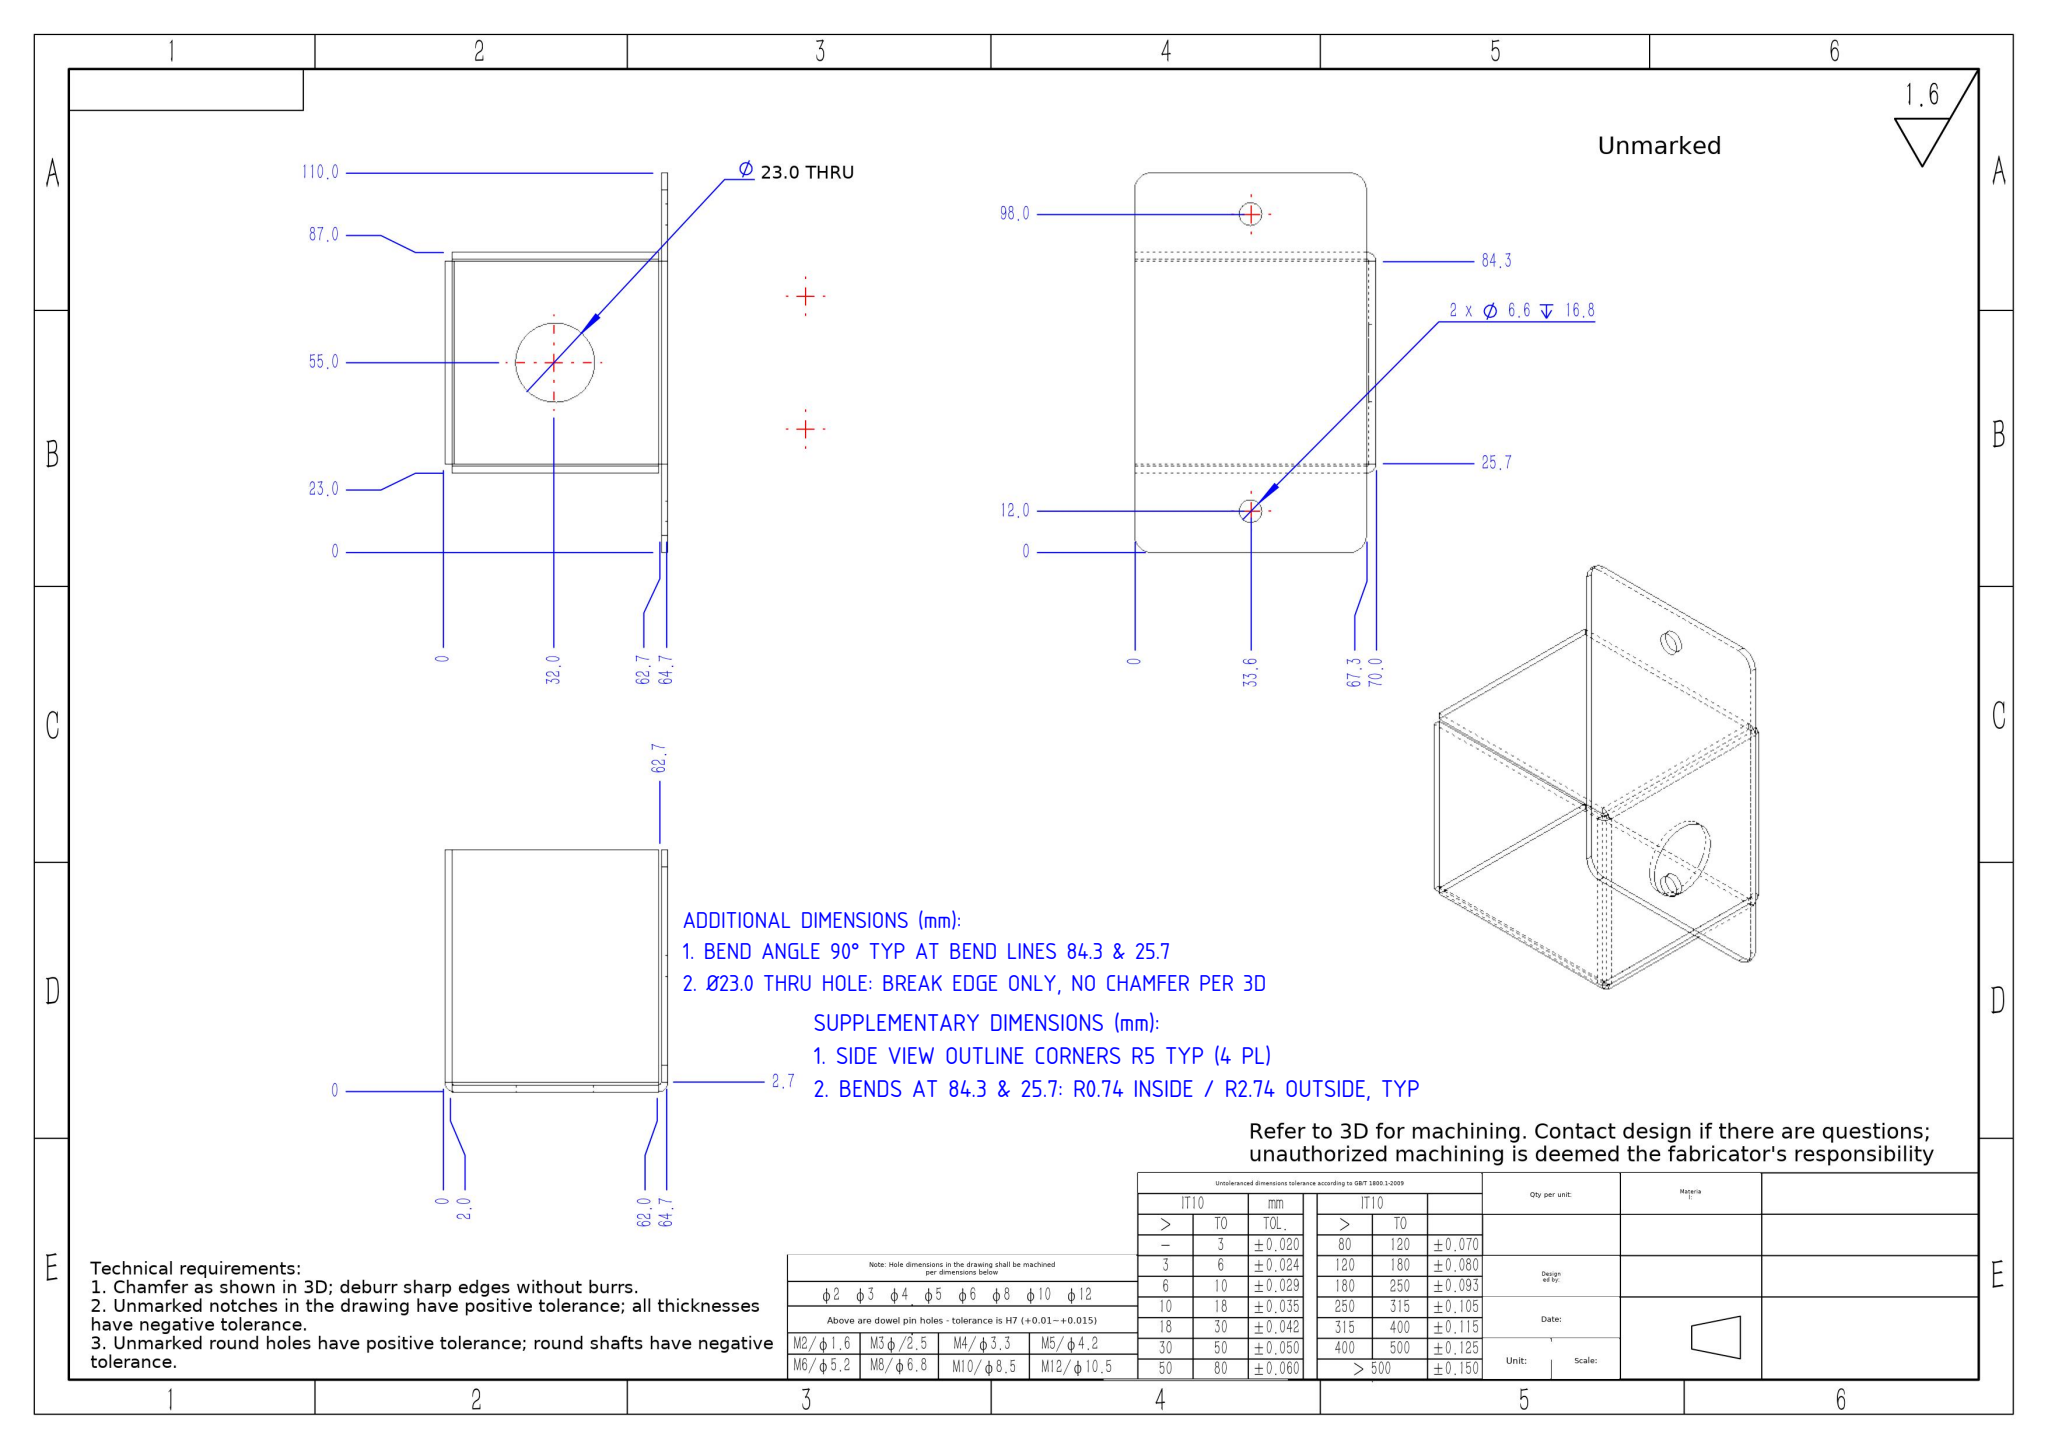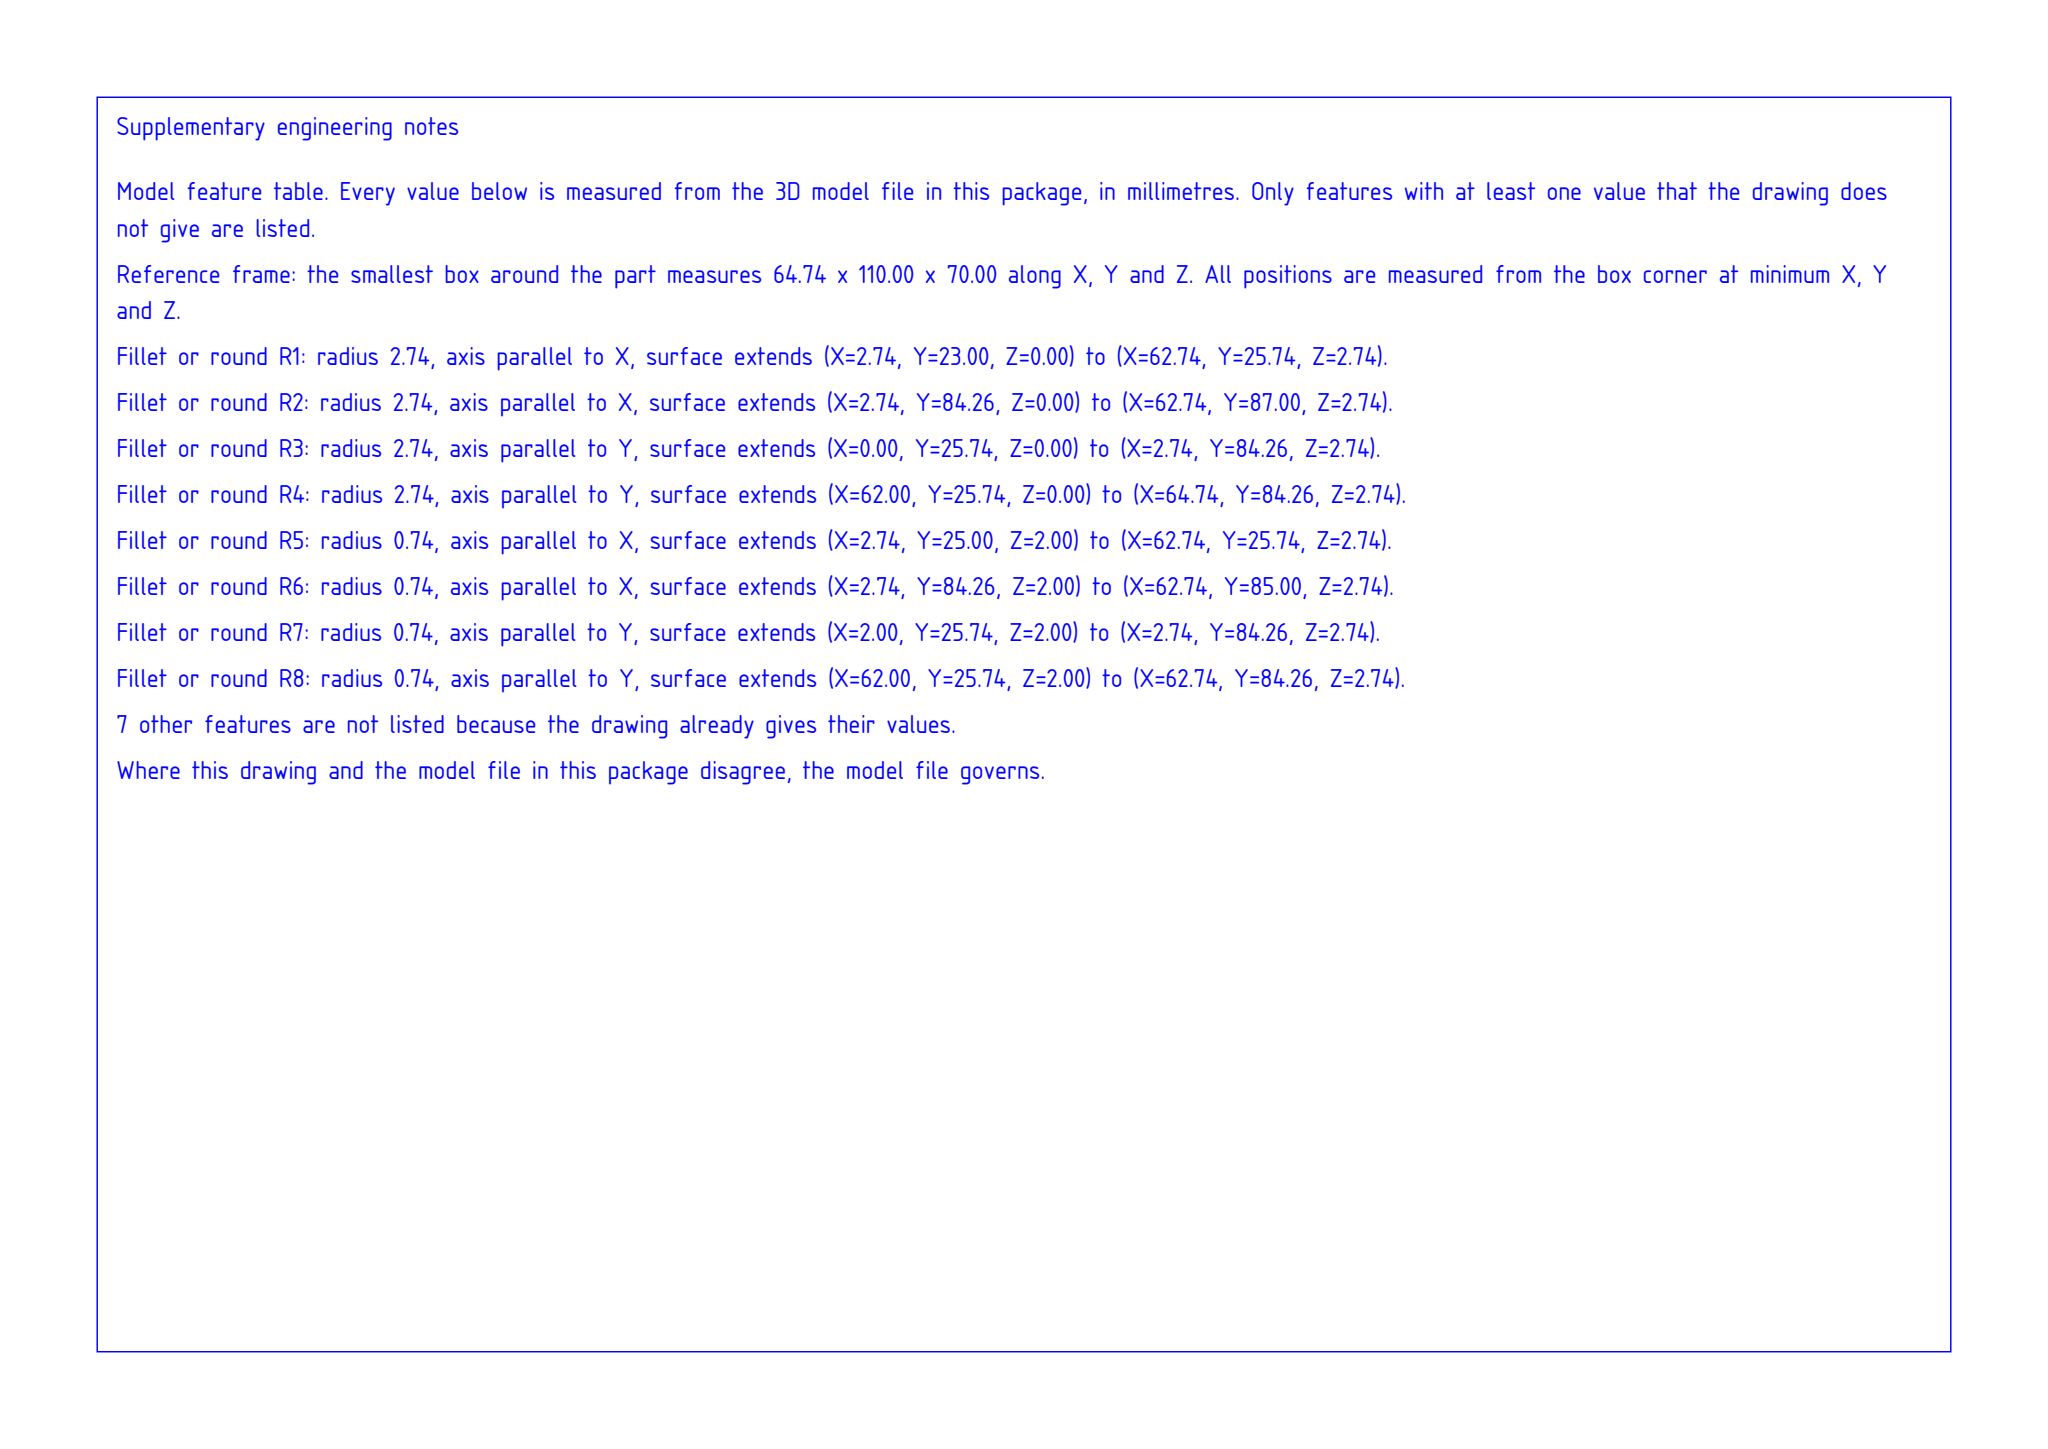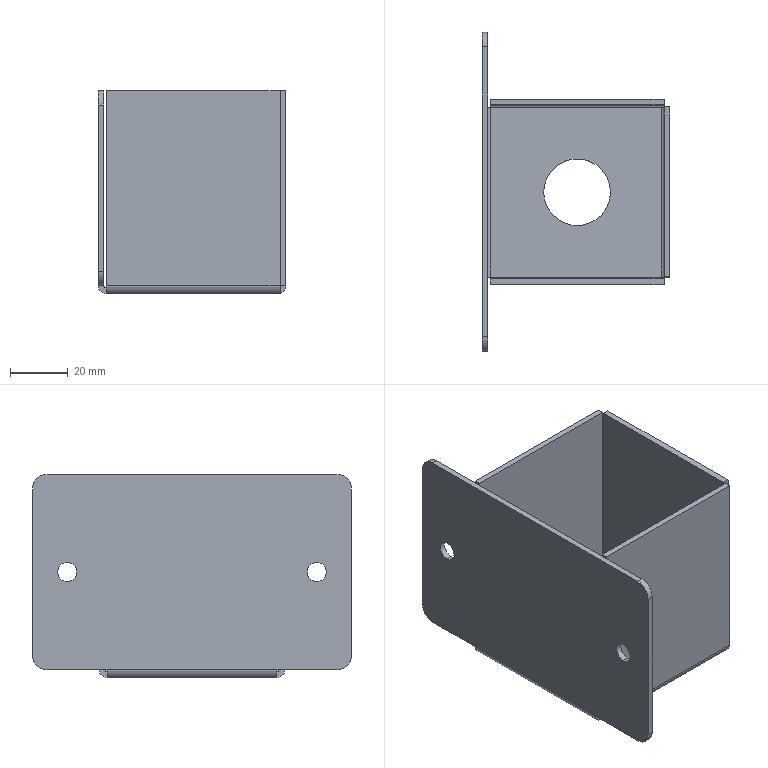Part | SolidWorks | mm | 1 solid | 52 faces | box 64.74 x 110 x 70 mm | volume 46034 mm3 | plane 34 | cylinder 18 | commonest cylinder face diameters 6.6 x4 5.473 x4 1.473 x4 10 x4 23 x2